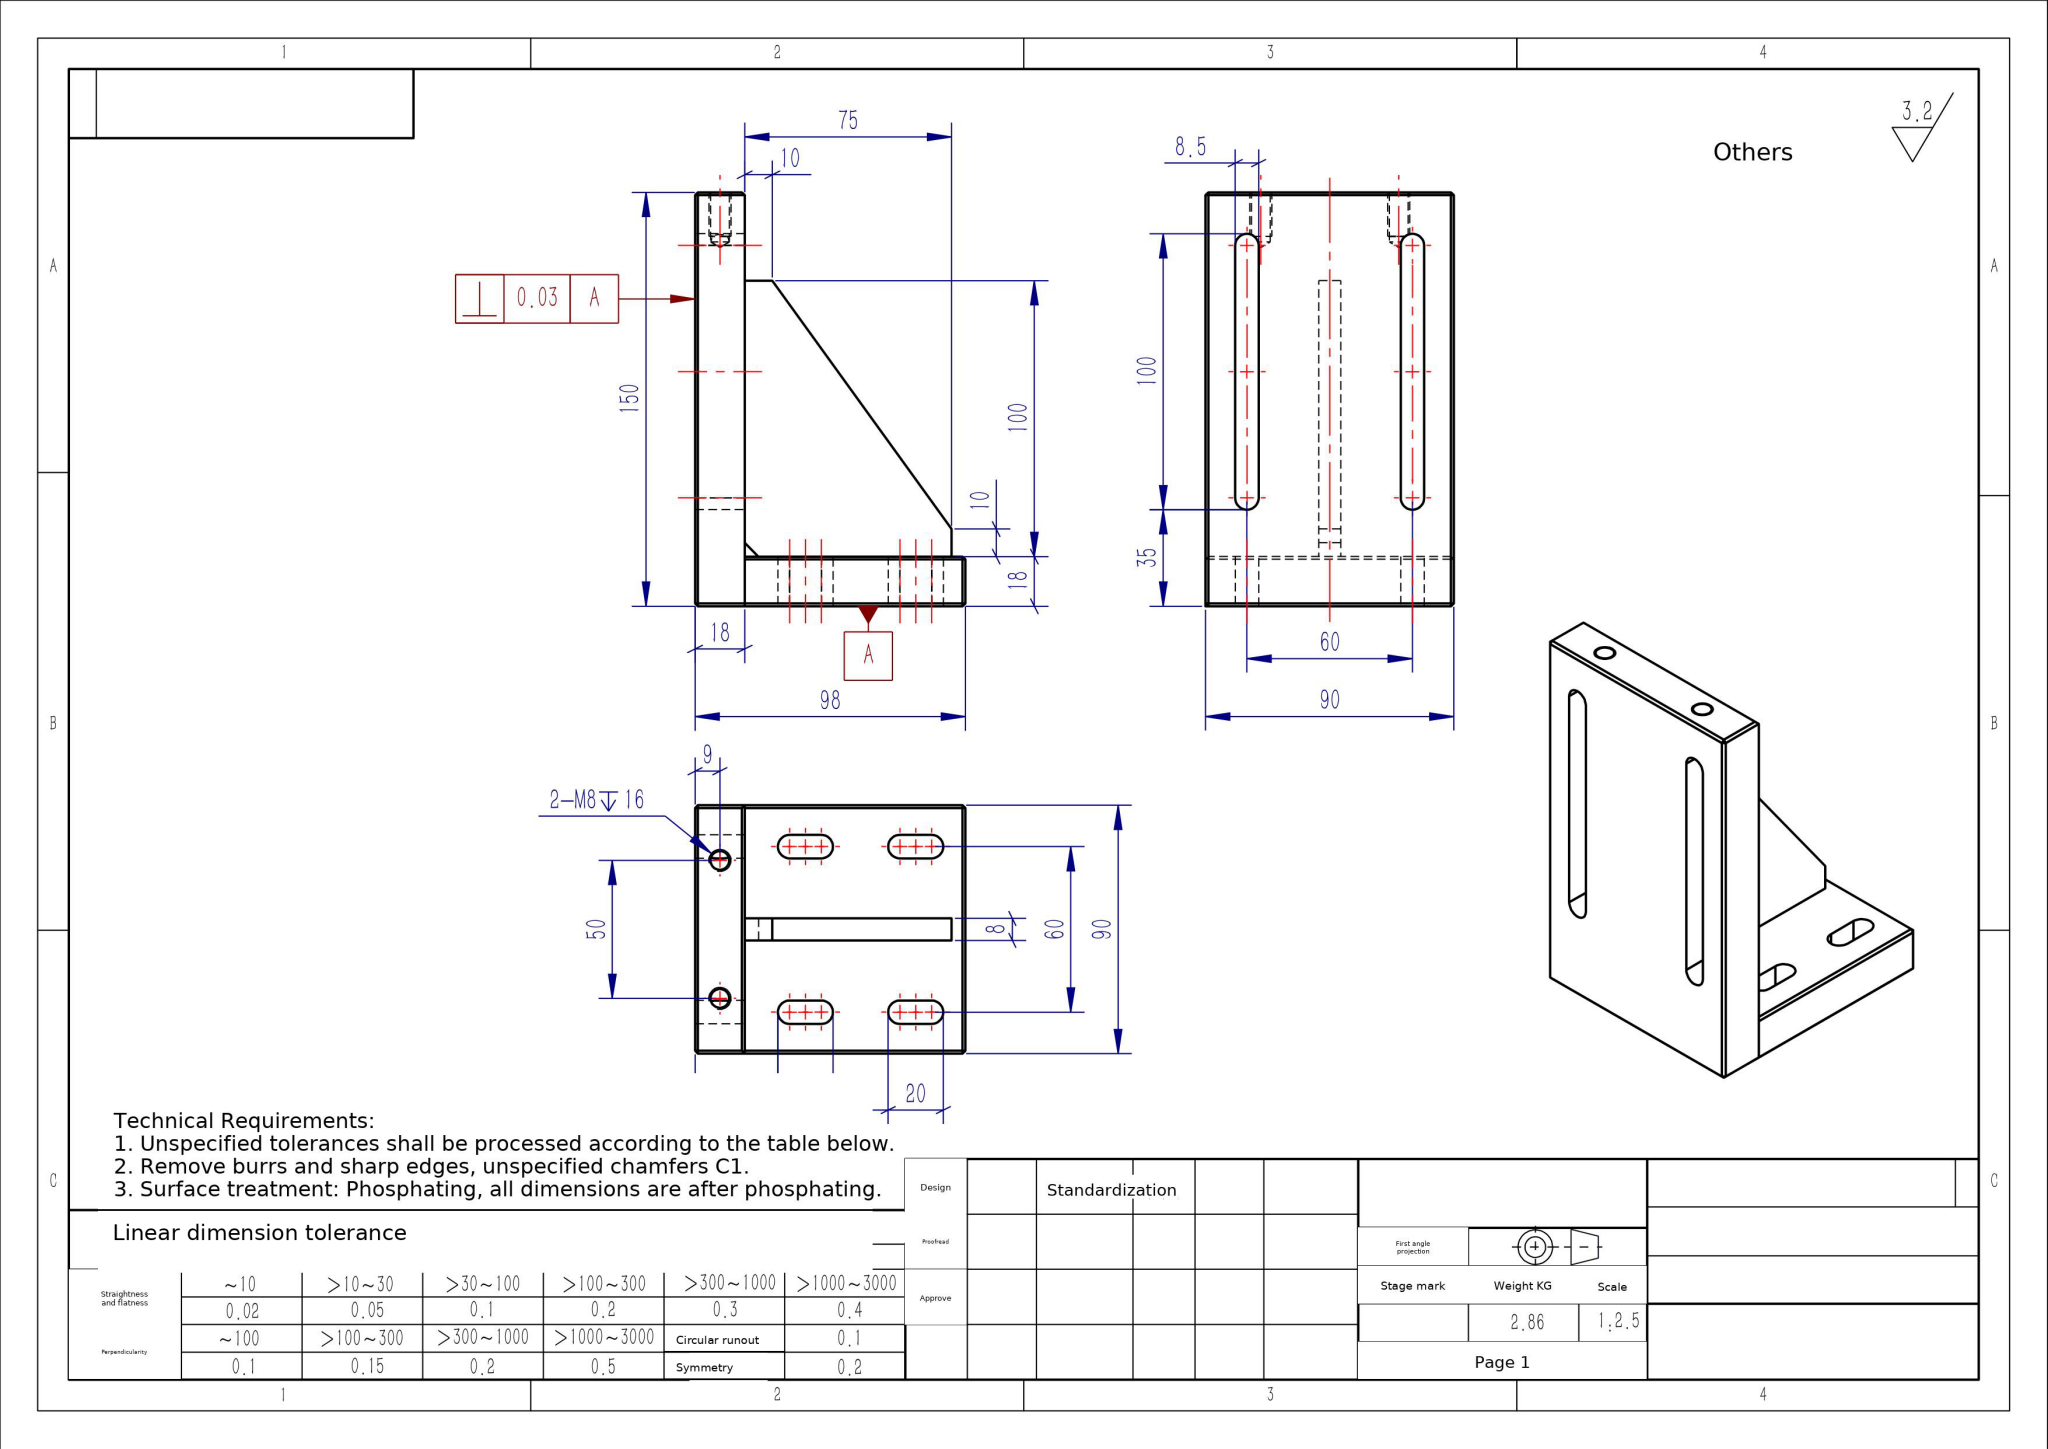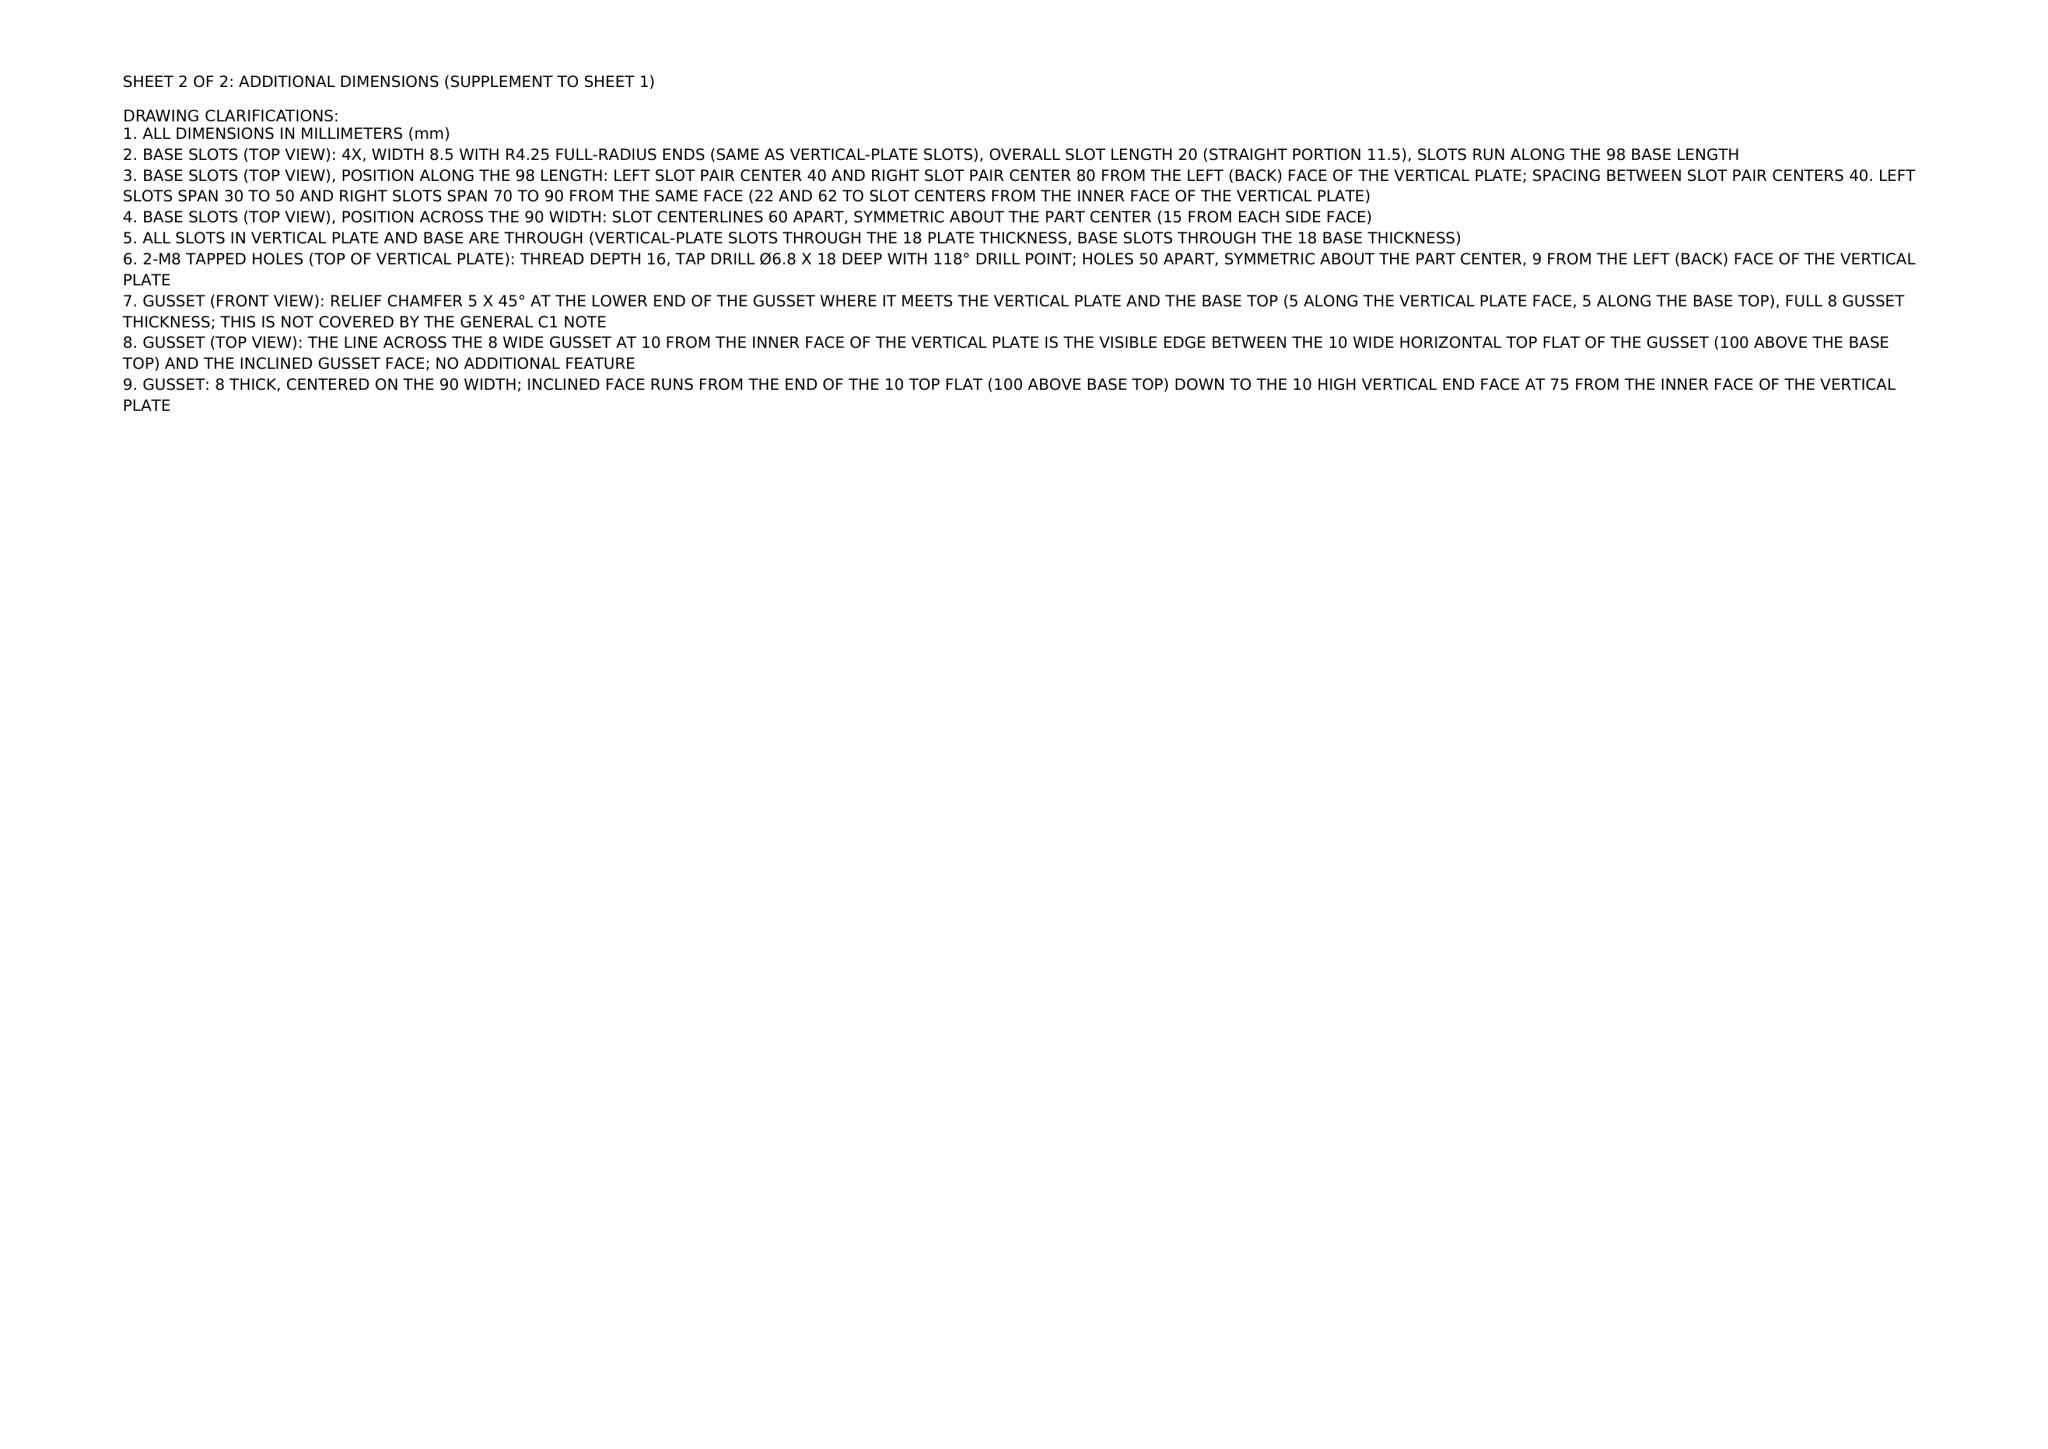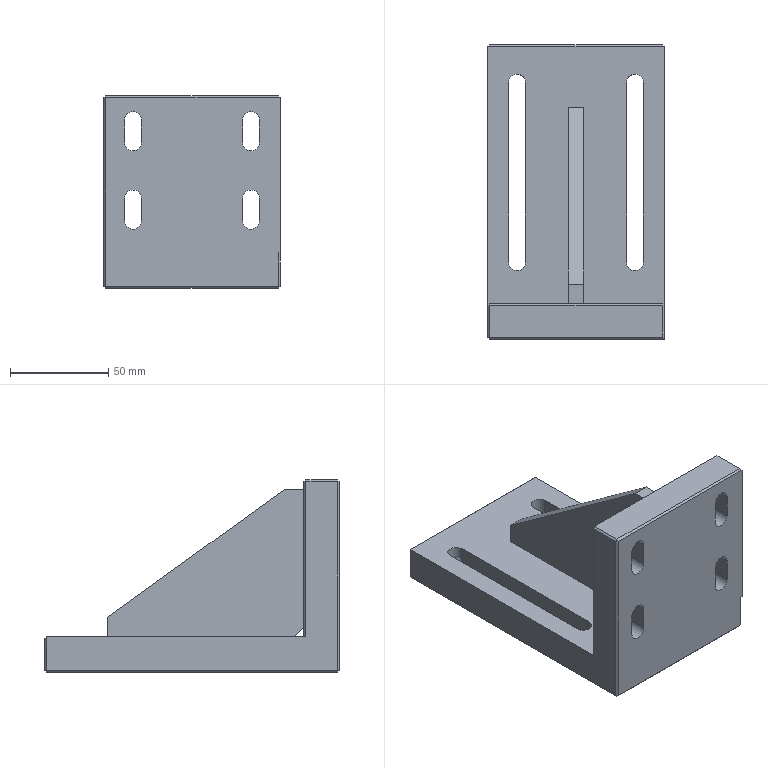Part | NX | mm | 1 solid | 73 faces | box 90 x 150 x 98 mm | volume 366106 mm3 | plane 49 | cylinder 20 | cone 4 | commonest cylinder face diameters 8.5 x16 6.8 x4